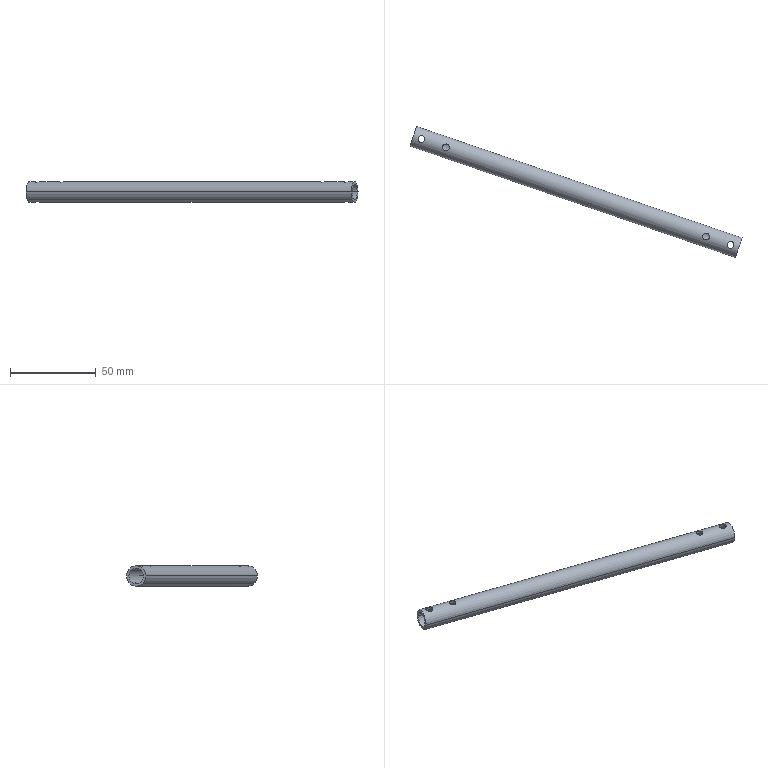Component | SolidWorks | ConnectingRod-1 | 1 solid | 18 faces | volume 9781 mm3 | cylinder 16 | plane 2 | commonest cylinder face diameters 4 x12 9 x2 12 x2